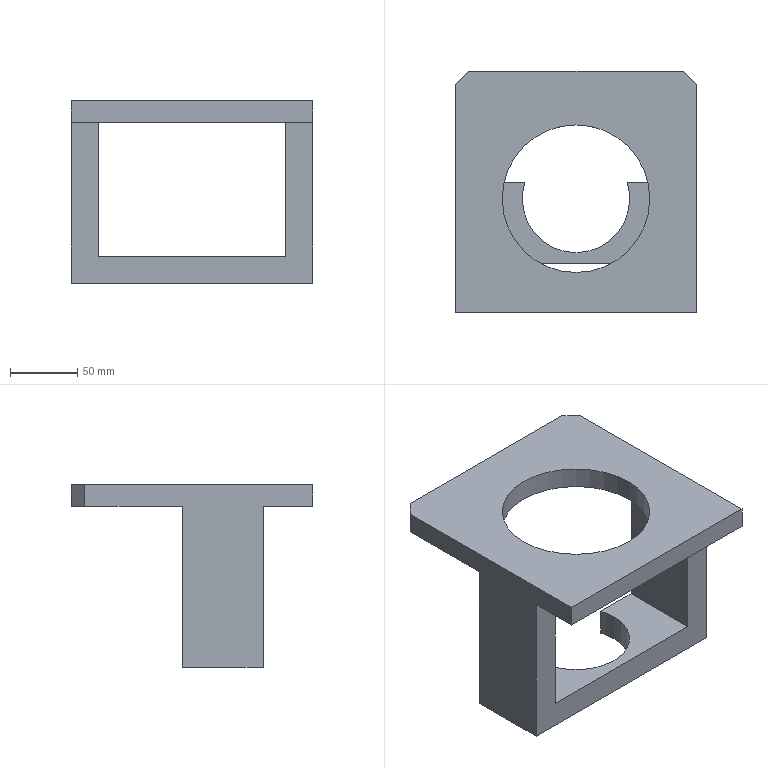Component | SolidWorks | L-Bracket-1 | 1 solid | 20 faces | box 180 x 180 x 136 mm | volume 751573 mm3 | plane 15 | cylinder 5 | commonest cylinder face diameters 80 x3 110 x2
build123d program:
from build123d import *

# Parameters (mm, degrees)
EXTRUDE1_DEPTH      = 90
CHAMFER1_SIZE       = 10
SKETCH3_R           = 55
CUT_EXTRUDE1_DEPTH  = 20
BOSS_EXTRUDE1_DEPTH = 60
SKETCH5_R           = 40
CUT_EXTRUDE2_DEPTH  = 230.87


with BuildPart() as part:
    # Sketch1 → Extrude1 (new, symmetric)
    with BuildSketch(Plane.XY):
        Polygon((0, 0), (0, -18), (16, -18), (16, -4), (16, 162), (0, 162), align=None)
    extrude(amount=EXTRUDE1_DEPTH, both=True)

    # Chamfer1
    chamfer1_edges = [part.edges().sort_by_distance(p)[0] for p in [
        (8, 162, 90),
        (8, 162, -90),
    ]]
    chamfer(chamfer1_edges, length=CHAMFER1_SIZE)

    # Sketch3 → Cut-Extrude1 (cut)
    with BuildSketch(Plane.ZY):
        with Locations((0, 67)):
            Circle(SKETCH3_R)
    extrude(amount=-CUT_EXTRUDE1_DEPTH, mode=Mode.SUBTRACT)

    # Sketch4 → Boss-Extrude1 (add)
    with BuildSketch(Plane.XZ.offset(-19)):
        Polygon((-120, -70), (-120, 70), (-120, 90), (0, 90), (0, 70), (-100, 70), (-100, -70), (0, -70), (0, -90), (-120, -90), align=None)
    extrude(amount=-BOSS_EXTRUDE1_DEPTH)

    # Sketch5 → Cut-Extrude2 (cut, through all)
    with BuildSketch(Plane(origin=(16, 0, 0), x_dir=(0, 0, -1), z_dir=(1, 0, 0))):
        with Locations((0, 67)):
            Circle(SKETCH5_R)
    extrude(amount=-CUT_EXTRUDE2_DEPTH, mode=Mode.SUBTRACT)


solid = part.part

# Placed as in the assembly
solid = solid.moved(Location((5.881, -63.556, 146), (0, -90, 0)))
STEP:
#1=COLOUR_RGB('',0.7922,0.8196,0.9333);
#2=FILL_AREA_STYLE_COLOUR('',#1);
#3=FILL_AREA_STYLE('',(#2));
#4=SURFACE_STYLE_FILL_AREA(#3);
#5=SURFACE_SIDE_STYLE('',(#4));
#6=SURFACE_STYLE_USAGE(.BOTH.,#5);
#7=PRESENTATION_STYLE_ASSIGNMENT((#6));
#8=CARTESIAN_POINT('',(-1.343,0.1356,1.024));
#9=VERTEX_POINT('',#8);
#10=CARTESIAN_POINT('',(1.806,0.1356,1.024));
#11=VERTEX_POINT('',#10);
#12=CARTESIAN_POINT('',(0.2315,0.1356,1.024));
#13=DIRECTION('',(0.,0.,1.));
#14=DIRECTION('',(1.,0.,0.));
#15=AXIS2_PLACEMENT_3D('',#12,#13,#14);
#16=CIRCLE('',#15,1.575);
#17=EDGE_CURVE('',#9,#11,#16,.T.);
#18=ORIENTED_EDGE('',*,*,#17,.F.);
#19=CARTESIAN_POINT('',(-1.343,0.1356,1.811));
#20=VERTEX_POINT('',#19);
#21=CARTESIAN_POINT('',(-1.343,0.1356,1.024));
#22=DIRECTION('',(0.,0.,1.));
#23=VECTOR('',#22,39.37);
#24=LINE('',#21,#23);
#25=EDGE_CURVE('',#9,#20,#24,.T.);
#26=ORIENTED_EDGE('',*,*,#25,.T.);
#27=CARTESIAN_POINT('',(1.806,0.1356,1.811));
#28=VERTEX_POINT('',#27);
#29=CARTESIAN_POINT('',(0.2315,0.1356,1.811));
#30=DIRECTION('',(-0.,0.,1.));
#31=DIRECTION('',(1.,0.,0.));
#32=AXIS2_PLACEMENT_3D('',#29,#30,#31);
#33=CIRCLE('',#32,1.575);
#34=EDGE_CURVE('',#20,#28,#33,.T.);
#35=ORIENTED_EDGE('',*,*,#34,.T.);
#36=CARTESIAN_POINT('',(1.806,0.1356,1.024));
#37=DIRECTION('',(0.,0.,1.));
#38=VECTOR('',#37,39.37);
#39=LINE('',#36,#38);
#40=EDGE_CURVE('',#11,#28,#39,.T.);
#41=ORIENTED_EDGE('',*,*,#40,.F.);
#42=EDGE_LOOP('',(#18,#26,#35,#41));
#43=FACE_OUTER_BOUND('',#42,.T.);
#44=CARTESIAN_POINT('',(0.2315,0.1356,1.024));
#45=DIRECTION('',(0.,0.,1.));
#46=DIRECTION('',(1.,0.,0.));
#47=AXIS2_PLACEMENT_3D('',#44,#45,#46);
#48=CYLINDRICAL_SURFACE('',#47,1.575);
#49=ADVANCED_FACE('',(#43),#48,.F.);
#50=CARTESIAN_POINT('',(1.734,0.608,1.024));
#51=VERTEX_POINT('',#50);
#52=CARTESIAN_POINT('',(0.2315,0.1356,1.024));
#53=DIRECTION('',(0.,0.,1.));
#54=DIRECTION('',(1.,0.,0.));
#55=AXIS2_PLACEMENT_3D('',#52,#53,#54);
#56=CIRCLE('',#55,1.575);
#57=EDGE_CURVE('',#11,#51,#56,.T.);
#58=ORIENTED_EDGE('',*,*,#57,.F.);
#59=ORIENTED_EDGE('',*,*,#40,.T.);
#60=CARTESIAN_POINT('',(1.734,0.608,1.811));
#61=VERTEX_POINT('',#60);
#62=CARTESIAN_POINT('',(0.2315,0.1356,1.811));
#63=DIRECTION('',(-0.,0.,1.));
#64=DIRECTION('',(1.,0.,0.));
#65=AXIS2_PLACEMENT_3D('',#62,#63,#64);
#66=CIRCLE('',#65,1.575);
#67=EDGE_CURVE('',#28,#61,#66,.T.);
#68=ORIENTED_EDGE('',*,*,#67,.T.);
#69=CARTESIAN_POINT('',(1.734,0.608,1.024));
#70=DIRECTION('',(0.,0.,-1.));
#71=VECTOR('',#70,39.37);
#72=LINE('',#69,#71);
#73=EDGE_CURVE('',#61,#51,#72,.T.);
#74=ORIENTED_EDGE('',*,*,#73,.T.);
#75=EDGE_LOOP('',(#58,#59,#68,#74));
#76=FACE_OUTER_BOUND('',#75,.T.);
#77=CARTESIAN_POINT('',(0.2315,0.1356,1.024));
#78=DIRECTION('',(0.,0.,1.));
#79=DIRECTION('',(1.,0.,0.));
#80=AXIS2_PLACEMENT_3D('',#77,#78,#79);
#81=CYLINDRICAL_SURFACE('',#80,1.575);
#82=ADVANCED_FACE('',(#76),#81,.F.);
#83=CARTESIAN_POINT('',(2.397,0.1356,6.378));
#84=VERTEX_POINT('',#83);
#85=CARTESIAN_POINT('',(-1.934,0.1356,6.378));
#86=VERTEX_POINT('',#85);
#87=CARTESIAN_POINT('',(0.2315,0.1356,6.378));
#88=DIRECTION('',(0.,0.,-1.));
#89=DIRECTION('',(-1.,0.,0.));
#90=AXIS2_PLACEMENT_3D('',#87,#88,#89);
#91=CIRCLE('',#90,2.165);
#92=EDGE_CURVE('',#84,#86,#91,.T.);
#93=ORIENTED_EDGE('',*,*,#92,.F.);
#94=CARTESIAN_POINT('',(2.397,0.1356,5.748));
#95=VERTEX_POINT('',#94);
#96=CARTESIAN_POINT('',(2.397,0.1356,6.535));
#97=DIRECTION('',(0.,0.,-1.));
#98=VECTOR('',#97,39.37);
#99=LINE('',#96,#98);
#100=EDGE_CURVE('',#84,#95,#99,.T.);
#101=ORIENTED_EDGE('',*,*,#100,.T.);
#102=CARTESIAN_POINT('',(-1.934,0.1356,5.748));
#103=VERTEX_POINT('',#102);
#104=CARTESIAN_POINT('',(0.2315,0.1356,5.748));
#105=DIRECTION('',(0.,0.,-1.));
#106=DIRECTION('',(-1.,0.,0.));
#107=AXIS2_PLACEMENT_3D('',#104,#105,#106);
#108=CIRCLE('',#107,2.165);
#109=EDGE_CURVE('',#95,#103,#108,.T.);
#110=ORIENTED_EDGE('',*,*,#109,.T.);
#111=CARTESIAN_POINT('',(-1.934,0.1356,6.535));
#112=DIRECTION('',(0.,0.,-1.));
#113=VECTOR('',#112,39.37);
#114=LINE('',#111,#113);
#115=EDGE_CURVE('',#86,#103,#114,.T.);
#116=ORIENTED_EDGE('',*,*,#115,.F.);
#117=EDGE_LOOP('',(#93,#101,#110,#116));
#118=FACE_OUTER_BOUND('',#117,.T.);
#119=CARTESIAN_POINT('',(0.2315,0.1356,6.535));
#120=DIRECTION('',(0.,0.,-1.));
#121=DIRECTION('',(-1.,0.,0.));
#122=AXIS2_PLACEMENT_3D('',#119,#120,#121);
#123=CYLINDRICAL_SURFACE('',#122,2.165);
#124=ADVANCED_FACE('',(#118),#123,.F.);
#125=CARTESIAN_POINT('',(-1.271,0.608,1.024));
#126=VERTEX_POINT('',#125);
#127=CARTESIAN_POINT('',(-1.271,0.608,1.811));
#128=VERTEX_POINT('',#127);
#129=CARTESIAN_POINT('',(-1.271,0.608,1.024));
#130=DIRECTION('',(0.,0.,1.));
#131=VECTOR('',#130,39.37);
#132=LINE('',#129,#131);
#133=EDGE_CURVE('',#126,#128,#132,.T.);
#134=ORIENTED_EDGE('',*,*,#133,.F.);
#135=CARTESIAN_POINT('',(-3.312,0.608,1.024));
#136=VERTEX_POINT('',#135);
#137=CARTESIAN_POINT('',(-3.312,0.608,1.024));
#138=DIRECTION('',(1.,0.,0.));
#139=VECTOR('',#138,39.37);
#140=LINE('',#137,#139);
#141=EDGE_CURVE('',#136,#126,#140,.T.);
#142=ORIENTED_EDGE('',*,*,#141,.F.);
#143=CARTESIAN_POINT('',(-3.312,0.608,5.748));
#144=VERTEX_POINT('',#143);
#145=CARTESIAN_POINT('',(-3.312,0.608,5.748));
#146=DIRECTION('',(0.,0.,-1.));
#147=VECTOR('',#146,39.37);
#148=LINE('',#145,#147);
#149=EDGE_CURVE('',#144,#136,#148,.T.);
#150=ORIENTED_EDGE('',*,*,#149,.F.);
#151=CARTESIAN_POINT('',(-2.524,0.608,5.748));
#152=VERTEX_POINT('',#151);
#153=CARTESIAN_POINT('',(-3.312,0.608,5.748));
#154=DIRECTION('',(-1.,0.,-0.));
#155=VECTOR('',#154,39.37);
#156=LINE('',#153,#155);
#157=EDGE_CURVE('',#152,#144,#156,.T.);
#158=ORIENTED_EDGE('',*,*,#157,.F.);
#159=CARTESIAN_POINT('',(-2.524,0.608,1.811));
#160=VERTEX_POINT('',#159);
#161=CARTESIAN_POINT('',(-2.524,0.608,5.748));
#162=DIRECTION('',(-0.,0.,1.));
#163=VECTOR('',#162,39.37);
#164=LINE('',#161,#163);
#165=EDGE_CURVE('',#160,#152,#164,.T.);
#166=ORIENTED_EDGE('',*,*,#165,.F.);
#167=CARTESIAN_POINT('',(-2.524,0.608,1.811));
#168=DIRECTION('',(-1.,0.,-0.));
#169=VECTOR('',#168,39.37);
#170=LINE('',#167,#169);
#171=EDGE_CURVE('',#128,#160,#170,.T.);
#172=ORIENTED_EDGE('',*,*,#171,.F.);
#173=EDGE_LOOP('',(#134,#142,#150,#158,#166,#172));
#174=FACE_OUTER_BOUND('',#173,.T.);
#175=CARTESIAN_POINT('',(-2.524,0.608,5.748));
#176=DIRECTION('',(0.,1.,0.));
#177=DIRECTION('',(-1.,0.,0.));
#178=AXIS2_PLACEMENT_3D('',#175,#176,#177);
#179=PLANE('',#178);
#180=ADVANCED_FACE('',(#174),#179,.T.);
#181=CARTESIAN_POINT('',(0.2315,0.1356,5.748));
#182=DIRECTION('',(0.,0.,-1.));
#183=DIRECTION('',(-1.,0.,0.));
#184=AXIS2_PLACEMENT_3D('',#181,#182,#183);
#185=CIRCLE('',#184,2.165);
#186=EDGE_CURVE('',#103,#95,#185,.T.);
#187=ORIENTED_EDGE('',*,*,#186,.F.);
#188=ORIENTED_EDGE('',*,*,#109,.F.);
#189=EDGE_LOOP('',(#187,#188));
#190=FACE_BOUND('',#189,.T.);
#191=CARTESIAN_POINT('',(3.775,3.482,5.748));
#192=VERTEX_POINT('',#191);
#193=CARTESIAN_POINT('',(3.775,0.608,5.748));
#194=VERTEX_POINT('',#193);
#195=CARTESIAN_POINT('',(3.775,-2.502,5.748));
#196=DIRECTION('',(0.,-1.,0.));
#197=VECTOR('',#196,39.37);
#198=LINE('',#195,#197);
#199=EDGE_CURVE('',#192,#194,#198,.T.);
#200=ORIENTED_EDGE('',*,*,#199,.T.);
#201=CARTESIAN_POINT('',(2.987,0.608,5.748));
#202=VERTEX_POINT('',#201);
#203=CARTESIAN_POINT('',(3.775,0.608,5.748));
#204=DIRECTION('',(-1.,0.,0.));
#205=VECTOR('',#204,39.37);
#206=LINE('',#203,#205);
#207=EDGE_CURVE('',#194,#202,#206,.T.);
#208=ORIENTED_EDGE('',*,*,#207,.T.);
#209=CARTESIAN_POINT('',(2.987,-1.754,5.748));
#210=VERTEX_POINT('',#209);
#211=CARTESIAN_POINT('',(2.987,0.608,5.748));
#212=DIRECTION('',(0.,-1.,0.));
#213=VECTOR('',#212,39.37);
#214=LINE('',#211,#213);
#215=EDGE_CURVE('',#202,#210,#214,.T.);
#216=ORIENTED_EDGE('',*,*,#215,.T.);
#217=CARTESIAN_POINT('',(3.775,-1.754,5.748));
#218=VERTEX_POINT('',#217);
#219=CARTESIAN_POINT('',(3.775,-1.754,5.748));
#220=DIRECTION('',(-1.,0.,0.));
#221=VECTOR('',#220,39.37);
#222=LINE('',#219,#221);
#223=EDGE_CURVE('',#218,#210,#222,.T.);
#224=ORIENTED_EDGE('',*,*,#223,.F.);
#225=CARTESIAN_POINT('',(3.775,-3.211,5.748));
#226=VERTEX_POINT('',#225);
#227=CARTESIAN_POINT('',(3.775,-2.502,5.748));
#228=DIRECTION('',(0.,-1.,0.));
#229=VECTOR('',#228,39.37);
#230=LINE('',#227,#229);
#231=EDGE_CURVE('',#218,#226,#230,.T.);
#232=ORIENTED_EDGE('',*,*,#231,.T.);
#233=CARTESIAN_POINT('',(-3.312,-3.211,5.748));
#234=VERTEX_POINT('',#233);
#235=CARTESIAN_POINT('',(-3.312,-3.211,5.748));
#236=DIRECTION('',(1.,0.,0.));
#237=VECTOR('',#236,39.37);
#238=LINE('',#235,#237);
#239=EDGE_CURVE('',#234,#226,#238,.T.);
#240=ORIENTED_EDGE('',*,*,#239,.F.);
#241=CARTESIAN_POINT('',(-3.312,-1.754,5.748));
#242=VERTEX_POINT('',#241);
#243=CARTESIAN_POINT('',(-3.312,-2.502,5.748));
#244=DIRECTION('',(0.,-1.,0.));
#245=VECTOR('',#244,39.37);
#246=LINE('',#243,#245);
#247=EDGE_CURVE('',#242,#234,#246,.T.);
#248=ORIENTED_EDGE('',*,*,#247,.F.);
#249=CARTESIAN_POINT('',(-2.524,-1.754,5.748));
#250=VERTEX_POINT('',#249);
#251=CARTESIAN_POINT('',(-3.312,-1.754,5.748));
#252=DIRECTION('',(-1.,0.,-0.));
#253=VECTOR('',#252,39.37);
#254=LINE('',#251,#253);
#255=EDGE_CURVE('',#250,#242,#254,.T.);
#256=ORIENTED_EDGE('',*,*,#255,.F.);
#257=CARTESIAN_POINT('',(-2.524,0.608,5.748));
#258=DIRECTION('',(0.,-1.,0.));
#259=VECTOR('',#258,39.37);
#260=LINE('',#257,#259);
#261=EDGE_CURVE('',#152,#250,#260,.T.);
#262=ORIENTED_EDGE('',*,*,#261,.F.);
#263=ORIENTED_EDGE('',*,*,#157,.T.);
#264=CARTESIAN_POINT('',(-3.312,3.482,5.748));
#265=VERTEX_POINT('',#264);
#266=CARTESIAN_POINT('',(-3.312,-2.502,5.748));
#267=DIRECTION('',(0.,-1.,0.));
#268=VECTOR('',#267,39.37);
#269=LINE('',#266,#268);
#270=EDGE_CURVE('',#265,#144,#269,.T.);
#271=ORIENTED_EDGE('',*,*,#270,.F.);
#272=CARTESIAN_POINT('',(-2.918,3.876,5.748));
#273=VERTEX_POINT('',#272);
#274=CARTESIAN_POINT('',(-3.312,3.482,5.748));
#275=DIRECTION('',(0.7071,0.7071,0.));
#276=VECTOR('',#275,39.37);
#277=LINE('',#274,#276);
#278=EDGE_CURVE('',#265,#273,#277,.T.);
#279=ORIENTED_EDGE('',*,*,#278,.T.);
#280=CARTESIAN_POINT('',(3.381,3.876,5.748));
#281=VERTEX_POINT('',#280);
#282=CARTESIAN_POINT('',(-3.312,3.876,5.748));
#283=DIRECTION('',(1.,0.,0.));
#284=VECTOR('',#283,39.37);
#285=LINE('',#282,#284);
#286=EDGE_CURVE('',#273,#281,#285,.T.);
#287=ORIENTED_EDGE('',*,*,#286,.T.);
#288=CARTESIAN_POINT('',(3.381,3.876,5.748));
#289=DIRECTION('',(0.7071,-0.7071,0.));
#290=VECTOR('',#289,39.37);
#291=LINE('',#288,#290);
#292=EDGE_CURVE('',#281,#192,#291,.T.);
#293=ORIENTED_EDGE('',*,*,#292,.T.);
#294=EDGE_LOOP('',(#200,#208,#216,#224,#232,#240,#248,#256,#262,#263,#271,#279,#287,#293));
#295=FACE_OUTER_BOUND('',#294,.T.);
#296=CARTESIAN_POINT('',(-3.312,-2.502,5.748));
#297=DIRECTION('',(0.,0.,1.));
#298=DIRECTION('',(1.,0.,0.));
#299=AXIS2_PLACEMENT_3D('',#296,#297,#298);
#300=PLANE('',#299);
#301=ADVANCED_FACE('',(#190,#295),#300,.F.);
#302=CARTESIAN_POINT('',(3.775,-3.211,6.378));
#303=VERTEX_POINT('',#302);
#304=CARTESIAN_POINT('',(3.775,-3.211,5.748));
#305=DIRECTION('',(0.,0.,1.));
#306=VECTOR('',#305,39.37);
#307=LINE('',#304,#306);
#308=EDGE_CURVE('',#226,#303,#307,.T.);
#309=ORIENTED_EDGE('',*,*,#308,.T.);
#310=CARTESIAN_POINT('',(-3.312,-3.211,6.378));
#311=VERTEX_POINT('',#310);
#312=CARTESIAN_POINT('',(-3.312,-3.211,6.378));
#313=DIRECTION('',(1.,0.,0.));
#314=VECTOR('',#313,39.37);
#315=LINE('',#312,#314);
#316=EDGE_CURVE('',#311,#303,#315,.T.);
#317=ORIENTED_EDGE('',*,*,#316,.F.);
#318=CARTESIAN_POINT('',(-3.312,-3.211,5.748));
#319=DIRECTION('',(0.,0.,1.));
#320=VECTOR('',#319,39.37);
#321=LINE('',#318,#320);
#322=EDGE_CURVE('',#234,#311,#321,.T.);
#323=ORIENTED_EDGE('',*,*,#322,.F.);
#324=ORIENTED_EDGE('',*,*,#239,.T.);
#325=EDGE_LOOP('',(#309,#317,#323,#324));
#326=FACE_OUTER_BOUND('',#325,.T.);
#327=CARTESIAN_POINT('',(-3.312,-3.211,5.748));
#328=DIRECTION('',(0.,1.,0.));
#329=DIRECTION('',(-1.,0.,0.));
#330=AXIS2_PLACEMENT_3D('',#327,#328,#329);
#331=PLANE('',#330);
#332=ADVANCED_FACE('',(#326),#331,.F.);
#333=CARTESIAN_POINT('',(0.2315,0.1356,6.378));
#334=DIRECTION('',(0.,0.,-1.));
#335=DIRECTION('',(-1.,0.,0.));
#336=AXIS2_PLACEMENT_3D('',#333,#334,#335);
#337=CIRCLE('',#336,2.165);
#338=EDGE_CURVE('',#86,#84,#337,.T.);
#339=ORIENTED_EDGE('',*,*,#338,.T.);
#340=ORIENTED_EDGE('',*,*,#92,.T.);
#341=EDGE_LOOP('',(#339,#340));
#342=FACE_BOUND('',#341,.T.);
#343=CARTESIAN_POINT('',(3.775,3.482,6.378));
#344=VERTEX_POINT('',#343);
#345=CARTESIAN_POINT('',(3.775,-2.66,6.378));
#346=DIRECTION('',(0.,1.,0.));
#347=VECTOR('',#346,39.37);
#348=LINE('',#345,#347);
#349=EDGE_CURVE('',#303,#344,#348,.T.);
#350=ORIENTED_EDGE('',*,*,#349,.T.);
#351=CARTESIAN_POINT('',(3.381,3.876,6.378));
#352=VERTEX_POINT('',#351);
#353=CARTESIAN_POINT('',(3.381,3.876,6.378));
#354=DIRECTION('',(-0.7071,0.7071,0.));
#355=VECTOR('',#354,39.37);
#356=LINE('',#353,#355);
#357=EDGE_CURVE('',#344,#352,#356,.T.);
#358=ORIENTED_EDGE('',*,*,#357,.T.);
#359=CARTESIAN_POINT('',(-2.918,3.876,6.378));
#360=VERTEX_POINT('',#359);
#361=CARTESIAN_POINT('',(-3.312,3.876,6.378));
#362=DIRECTION('',(1.,0.,0.));
#363=VECTOR('',#362,39.37);
#364=LINE('',#361,#363);
#365=EDGE_CURVE('',#360,#352,#364,.T.);
#366=ORIENTED_EDGE('',*,*,#365,.F.);
#367=CARTESIAN_POINT('',(-3.312,3.482,6.378));
#368=VERTEX_POINT('',#367);
#369=CARTESIAN_POINT('',(-3.312,3.482,6.378));
#370=DIRECTION('',(-0.7071,-0.7071,0.));
#371=VECTOR('',#370,39.37);
#372=LINE('',#369,#371);
#373=EDGE_CURVE('',#360,#368,#372,.T.);
#374=ORIENTED_EDGE('',*,*,#373,.T.);
#375=CARTESIAN_POINT('',(-3.312,-2.66,6.378));
#376=DIRECTION('',(0.,1.,0.));
#377=VECTOR('',#376,39.37);
#378=LINE('',#375,#377);
#379=EDGE_CURVE('',#311,#368,#378,.T.);
#380=ORIENTED_EDGE('',*,*,#379,.F.);
#381=ORIENTED_EDGE('',*,*,#316,.T.);
#382=EDGE_LOOP('',(#350,#358,#366,#374,#380,#381));
#383=FACE_OUTER_BOUND('',#382,.T.);
#384=CARTESIAN_POINT('',(-3.312,-2.66,6.378));
#385=DIRECTION('',(0.,0.,-1.));
#386=DIRECTION('',(-1.,0.,0.));
#387=AXIS2_PLACEMENT_3D('',#384,#385,#386);
#388=PLANE('',#387);
#389=ADVANCED_FACE('',(#342,#383),#388,.F.);
#390=ORIENTED_EDGE('',*,*,#365,.T.);
#391=CARTESIAN_POINT('',(3.381,3.876,5.748));
#392=DIRECTION('',(0.,0.,-1.));
#393=VECTOR('',#392,39.37);
#394=LINE('',#391,#393);
#395=EDGE_CURVE('',#352,#281,#394,.T.);
#396=ORIENTED_EDGE('',*,*,#395,.T.);
#397=ORIENTED_EDGE('',*,*,#286,.F.);
#398=CARTESIAN_POINT('',(-2.918,3.876,5.748));
#399=DIRECTION('',(0.,0.,1.));
#400=VECTOR('',#399,39.37);
#401=LINE('',#398,#400);
#402=EDGE_CURVE('',#273,#360,#401,.T.);
#403=ORIENTED_EDGE('',*,*,#402,.T.);
#404=EDGE_LOOP('',(#390,#396,#397,#403));
#405=FACE_OUTER_BOUND('',#404,.T.);
#406=CARTESIAN_POINT('',(-3.312,3.876,5.748));
#407=DIRECTION('',(0.,-1.,0.));
#408=DIRECTION('',(1.,0.,0.));
#409=AXIS2_PLACEMENT_3D('',#406,#407,#408);
#410=PLANE('',#409);
#411=ADVANCED_FACE('',(#405),#410,.F.);
#412=ORIENTED_EDGE('',*,*,#379,.T.);
#413=CARTESIAN_POINT('',(-3.312,3.482,5.748));
#414=DIRECTION('',(0.,0.,-1.));
#415=VECTOR('',#414,39.37);
#416=LINE('',#413,#415);
#417=EDGE_CURVE('',#368,#265,#416,.T.);
#418=ORIENTED_EDGE('',*,*,#417,.T.);
#419=ORIENTED_EDGE('',*,*,#270,.T.);
#420=ORIENTED_EDGE('',*,*,#149,.T.);
#421=CARTESIAN_POINT('',(-3.312,-1.754,1.024));
#422=VERTEX_POINT('',#421);
#423=CARTESIAN_POINT('',(-3.312,0.608,1.024));
#424=DIRECTION('',(0.,-1.,0.));
#425=VECTOR('',#424,39.37);
#426=LINE('',#423,#425);
#427=EDGE_CURVE('',#136,#422,#426,.T.);
#428=ORIENTED_EDGE('',*,*,#427,.T.);
#429=CARTESIAN_POINT('',(-3.312,-1.754,5.748));
#430=DIRECTION('',(0.,0.,-1.));
#431=VECTOR('',#430,39.37);
#432=LINE('',#429,#431);
#433=EDGE_CURVE('',#242,#422,#432,.T.);
#434=ORIENTED_EDGE('',*,*,#433,.F.);
#435=ORIENTED_EDGE('',*,*,#247,.T.);
#436=ORIENTED_EDGE('',*,*,#322,.T.);
#437=EDGE_LOOP('',(#412,#418,#419,#420,#428,#434,#435,#436));
#438=FACE_OUTER_BOUND('',#437,.T.);
#439=CARTESIAN_POINT('',(-3.312,3.876,5.748));
#440=DIRECTION('',(1.,0.,0.));
#441=DIRECTION('',(0.,0.,-1.));
#442=AXIS2_PLACEMENT_3D('',#439,#440,#441);
#443=PLANE('',#442);
#444=ADVANCED_FACE('',(#438),#443,.F.);
#445=ORIENTED_EDGE('',*,*,#199,.F.);
#446=CARTESIAN_POINT('',(3.775,3.482,6.378));
#447=DIRECTION('',(0.,0.,1.));
#448=VECTOR('',#447,39.37);
#449=LINE('',#446,#448);
#450=EDGE_CURVE('',#192,#344,#449,.T.);
#451=ORIENTED_EDGE('',*,*,#450,.T.);
#452=ORIENTED_EDGE('',*,*,#349,.F.);
#453=ORIENTED_EDGE('',*,*,#308,.F.);
#454=ORIENTED_EDGE('',*,*,#231,.F.);
#455=CARTESIAN_POINT('',(3.775,-1.754,1.024));
#456=VERTEX_POINT('',#455);
#457=CARTESIAN_POINT('',(3.775,-1.754,5.748));
#458=DIRECTION('',(-0.,0.,1.));
#459=VECTOR('',#458,39.37);
#460=LINE('',#457,#459);
#461=EDGE_CURVE('',#456,#218,#460,.T.);
#462=ORIENTED_EDGE('',*,*,#461,.F.);
#463=CARTESIAN_POINT('',(3.775,0.608,1.024));
#464=VERTEX_POINT('',#463);
#465=CARTESIAN_POINT('',(3.775,0.608,1.024));
#466=DIRECTION('',(0.,-1.,0.));
#467=VECTOR('',#466,39.37);
#468=LINE('',#465,#467);
#469=EDGE_CURVE('',#464,#456,#468,.T.);
#470=ORIENTED_EDGE('',*,*,#469,.F.);
#471=CARTESIAN_POINT('',(3.775,0.608,5.748));
#472=DIRECTION('',(-0.,0.,1.));
#473=VECTOR('',#472,39.37);
#474=LINE('',#471,#473);
#475=EDGE_CURVE('',#464,#194,#474,.T.);
#476=ORIENTED_EDGE('',*,*,#475,.T.);
#477=EDGE_LOOP('',(#445,#451,#452,#453,#454,#462,#470,#476));
#478=FACE_OUTER_BOUND('',#477,.T.);
#479=CARTESIAN_POINT('',(3.775,3.876,5.748));
#480=DIRECTION('',(1.,0.,0.));
#481=DIRECTION('',(0.,0.,-1.));
#482=AXIS2_PLACEMENT_3D('',#479,#480,#481);
#483=PLANE('',#482);
#484=ADVANCED_FACE('',(#478),#483,.T.);
#485=ORIENTED_EDGE('',*,*,#357,.F.);
#486=ORIENTED_EDGE('',*,*,#450,.F.);
#487=ORIENTED_EDGE('',*,*,#292,.F.);
#488=ORIENTED_EDGE('',*,*,#395,.F.);
#489=EDGE_LOOP('',(#485,#486,#487,#488));
#490=FACE_OUTER_BOUND('',#489,.T.);
#491=CARTESIAN_POINT('',(3.381,3.876,5.748));
#492=DIRECTION('',(0.7071,0.7071,0.));
#493=DIRECTION('',(-0.7071,0.7071,0.));
#494=AXIS2_PLACEMENT_3D('',#491,#492,#493);
#495=PLANE('',#494);
#496=ADVANCED_FACE('',(#490),#495,.T.);
#497=ORIENTED_EDGE('',*,*,#373,.F.);
#498=ORIENTED_EDGE('',*,*,#402,.F.);
#499=ORIENTED_EDGE('',*,*,#278,.F.);
#500=ORIENTED_EDGE('',*,*,#417,.F.);
#501=EDGE_LOOP('',(#497,#498,#499,#500));
#502=FACE_OUTER_BOUND('',#501,.T.);
#503=CARTESIAN_POINT('',(-3.312,3.482,5.748));
#504=DIRECTION('',(0.7071,-0.7071,0.));
#505=DIRECTION('',(0.7071,0.7071,0.));
#506=AXIS2_PLACEMENT_3D('',#503,#504,#505);
#507=PLANE('',#506);
#508=ADVANCED_FACE('',(#502),#507,.F.);
#509=ORIENTED_EDGE('',*,*,#100,.F.);
#510=ORIENTED_EDGE('',*,*,#338,.F.);
#511=ORIENTED_EDGE('',*,*,#115,.T.);
#512=ORIENTED_EDGE('',*,*,#186,.T.);
#513=EDGE_LOOP('',(#509,#510,#511,#512));
#514=FACE_OUTER_BOUND('',#513,.T.);
#515=CARTESIAN_POINT('',(0.2315,0.1356,6.535));
#516=DIRECTION('',(0.,0.,-1.));
#517=DIRECTION('',(-1.,0.,0.));
#518=AXIS2_PLACEMENT_3D('',#515,#516,#517);
#519=CYLINDRICAL_SURFACE('',#518,2.165);
#520=ADVANCED_FACE('',(#514),#519,.F.);
#521=CARTESIAN_POINT('',(-2.524,-1.754,1.811));
#522=VERTEX_POINT('',#521);
#523=CARTESIAN_POINT('',(-2.524,-1.754,5.748));
#524=DIRECTION('',(-0.,0.,1.));
#525=VECTOR('',#524,39.37);
#526=LINE('',#523,#525);
#527=EDGE_CURVE('',#522,#250,#526,.T.);
#528=ORIENTED_EDGE('',*,*,#527,.F.);
#529=CARTESIAN_POINT('',(-2.524,0.608,1.811));
#530=DIRECTION('',(0.,-1.,0.));
#531=VECTOR('',#530,39.37);
#532=LINE('',#529,#531);
#533=EDGE_CURVE('',#160,#522,#532,.T.);
#534=ORIENTED_EDGE('',*,*,#533,.F.);
#535=ORIENTED_EDGE('',*,*,#165,.T.);
#536=ORIENTED_EDGE('',*,*,#261,.T.);
#537=EDGE_LOOP('',(#528,#534,#535,#536));
#538=FACE_OUTER_BOUND('',#537,.T.);
#539=CARTESIAN_POINT('',(-2.524,0.608,5.748));
#540=DIRECTION('',(1.,0.,0.));
#541=DIRECTION('',(0.,0.,-1.));
#542=AXIS2_PLACEMENT_3D('',#539,#540,#541);
#543=PLANE('',#542);
#544=ADVANCED_FACE('',(#538),#543,.T.);
#545=CARTESIAN_POINT('',(0.2315,0.1356,1.811));
#546=DIRECTION('',(-0.,0.,1.));
#547=DIRECTION('',(1.,0.,0.));
#548=AXIS2_PLACEMENT_3D('',#545,#546,#547);
#549=CIRCLE('',#548,1.575);
#550=EDGE_CURVE('',#128,#20,#549,.T.);
#551=ORIENTED_EDGE('',*,*,#550,.F.);
#552=ORIENTED_EDGE('',*,*,#171,.T.);
#553=ORIENTED_EDGE('',*,*,#533,.T.);
#554=CARTESIAN_POINT('',(2.987,-1.754,1.811));
#555=VERTEX_POINT('',#554);
#556=CARTESIAN_POINT('',(-2.524,-1.754,1.811));
#557=DIRECTION('',(-1.,0.,-0.));
#558=VECTOR('',#557,39.37);
#559=LINE('',#556,#558);
#560=EDGE_CURVE('',#555,#522,#559,.T.);
#561=ORIENTED_EDGE('',*,*,#560,.F.);
#562=CARTESIAN_POINT('',(2.987,0.608,1.811));
#563=VERTEX_POINT('',#562);
#564=CARTESIAN_POINT('',(2.987,0.608,1.811));
#565=DIRECTION('',(0.,-1.,0.));
#566=VECTOR('',#565,39.37);
#567=LINE('',#564,#566);
#568=EDGE_CURVE('',#563,#555,#567,.T.);
#569=ORIENTED_EDGE('',*,*,#568,.F.);
#570=CARTESIAN_POINT('',(-2.524,0.608,1.811));
#571=DIRECTION('',(-1.,0.,-0.));
#572=VECTOR('',#571,39.37);
#573=LINE('',#570,#572);
#574=EDGE_CURVE('',#563,#61,#573,.T.);
#575=ORIENTED_EDGE('',*,*,#574,.T.);
#576=ORIENTED_EDGE('',*,*,#67,.F.);
#577=ORIENTED_EDGE('',*,*,#34,.F.);
#578=EDGE_LOOP('',(#551,#552,#553,#561,#569,#575,#576,#577));
#579=FACE_OUTER_BOUND('',#578,.T.);
#580=CARTESIAN_POINT('',(-2.524,0.608,1.811));
#581=DIRECTION('',(-0.,0.,1.));
#582=DIRECTION('',(1.,0.,0.));
#583=AXIS2_PLACEMENT_3D('',#580,#581,#582);
#584=PLANE('',#583);
#585=ADVANCED_FACE('',(#579),#584,.T.);
#586=CARTESIAN_POINT('',(2.987,-1.754,5.748));
#587=DIRECTION('',(0.,0.,-1.));
#588=VECTOR('',#587,39.37);
#589=LINE('',#586,#588);
#590=EDGE_CURVE('',#210,#555,#589,.T.);
#591=ORIENTED_EDGE('',*,*,#590,.F.);
#592=ORIENTED_EDGE('',*,*,#215,.F.);
#593=CARTESIAN_POINT('',(2.987,0.608,5.748));
#594=DIRECTION('',(0.,0.,-1.));
#595=VECTOR('',#594,39.37);
#596=LINE('',#593,#595);
#597=EDGE_CURVE('',#202,#563,#596,.T.);
#598=ORIENTED_EDGE('',*,*,#597,.T.);
#599=ORIENTED_EDGE('',*,*,#568,.T.);
#600=EDGE_LOOP('',(#591,#592,#598,#599));
#601=FACE_OUTER_BOUND('',#600,.T.);
#602=CARTESIAN_POINT('',(2.987,0.608,5.748));
#603=DIRECTION('',(-1.,0.,-0.));
#604=DIRECTION('',(-0.,0.,1.));
#605=AXIS2_PLACEMENT_3D('',#602,#603,#604);
#606=PLANE('',#605);
#607=ADVANCED_FACE('',(#601),#606,.T.);
#608=CARTESIAN_POINT('',(0.2315,0.1356,1.024));
#609=DIRECTION('',(0.,0.,1.));
#610=DIRECTION('',(1.,0.,0.));
#611=AXIS2_PLACEMENT_3D('',#608,#609,#610);
#612=CIRCLE('',#611,1.575);
#613=EDGE_CURVE('',#126,#9,#612,.T.);
#614=ORIENTED_EDGE('',*,*,#613,.T.);
#615=ORIENTED_EDGE('',*,*,#17,.T.);
#616=ORIENTED_EDGE('',*,*,#57,.T.);
#617=CARTESIAN_POINT('',(-3.312,0.608,1.024));
#618=DIRECTION('',(1.,0.,0.));
#619=VECTOR('',#618,39.37);
#620=LINE('',#617,#619);
#621=EDGE_CURVE('',#51,#464,#620,.T.);
#622=ORIENTED_EDGE('',*,*,#621,.T.);
#623=ORIENTED_EDGE('',*,*,#469,.T.);
#624=CARTESIAN_POINT('',(3.775,-1.754,1.024));
#625=DIRECTION('',(1.,0.,0.));
#626=VECTOR('',#625,39.37);
#627=LINE('',#624,#626);
#628=EDGE_CURVE('',#422,#456,#627,.T.);
#629=ORIENTED_EDGE('',*,*,#628,.F.);
#630=ORIENTED_EDGE('',*,*,#427,.F.);
#631=ORIENTED_EDGE('',*,*,#141,.T.);
#632=EDGE_LOOP('',(#614,#615,#616,#622,#623,#629,#630,#631));
#633=FACE_OUTER_BOUND('',#632,.T.);
#634=CARTESIAN_POINT('',(3.775,0.608,1.024));
#635=DIRECTION('',(0.,0.,-1.));
#636=DIRECTION('',(-1.,0.,0.));
#637=AXIS2_PLACEMENT_3D('',#634,#635,#636);
#638=PLANE('',#637);
#639=ADVANCED_FACE('',(#633),#638,.T.);
#640=ORIENTED_EDGE('',*,*,#73,.F.);
#641=ORIENTED_EDGE('',*,*,#574,.F.);
#642=ORIENTED_EDGE('',*,*,#597,.F.);
#643=ORIENTED_EDGE('',*,*,#207,.F.);
#644=ORIENTED_EDGE('',*,*,#475,.F.);
#645=ORIENTED_EDGE('',*,*,#621,.F.);
#646=EDGE_LOOP('',(#640,#641,#642,#643,#644,#645));
#647=FACE_OUTER_BOUND('',#646,.T.);
#648=CARTESIAN_POINT('',(-2.524,0.608,5.748));
#649=DIRECTION('',(0.,1.,0.));
#650=DIRECTION('',(-1.,0.,0.));
#651=AXIS2_PLACEMENT_3D('',#648,#649,#650);
#652=PLANE('',#651);
#653=ADVANCED_FACE('',(#647),#652,.T.);
#654=ORIENTED_EDGE('',*,*,#255,.T.);
#655=ORIENTED_EDGE('',*,*,#433,.T.);
#656=ORIENTED_EDGE('',*,*,#628,.T.);
#657=ORIENTED_EDGE('',*,*,#461,.T.);
#658=ORIENTED_EDGE('',*,*,#223,.T.);
#659=ORIENTED_EDGE('',*,*,#590,.T.);
#660=ORIENTED_EDGE('',*,*,#560,.T.);
#661=ORIENTED_EDGE('',*,*,#527,.T.);
#662=EDGE_LOOP('',(#654,#655,#656,#657,#658,#659,#660,#661));
#663=FACE_OUTER_BOUND('',#662,.T.);
#664=CARTESIAN_POINT('',(-2.524,-1.754,5.748));
#665=DIRECTION('',(0.,1.,0.));
#666=DIRECTION('',(-1.,0.,0.));
#667=AXIS2_PLACEMENT_3D('',#664,#665,#666);
#668=PLANE('',#667);
#669=ADVANCED_FACE('',(#663),#668,.F.);
#670=ORIENTED_EDGE('',*,*,#25,.F.);
#671=ORIENTED_EDGE('',*,*,#613,.F.);
#672=ORIENTED_EDGE('',*,*,#133,.T.);
#673=ORIENTED_EDGE('',*,*,#550,.T.);
#674=EDGE_LOOP('',(#670,#671,#672,#673));
#675=FACE_OUTER_BOUND('',#674,.T.);
#676=CARTESIAN_POINT('',(0.2315,0.1356,1.024));
#677=DIRECTION('',(0.,0.,1.));
#678=DIRECTION('',(1.,0.,0.));
#679=AXIS2_PLACEMENT_3D('',#676,#677,#678);
#680=CYLINDRICAL_SURFACE('',#679,1.575);
#681=ADVANCED_FACE('',(#675),#680,.F.);
#682=CLOSED_SHELL('',(#49,#82,#124,#180,#301,#332,#389,#411,#444,#484,#496,#508,#520,#544,#585,#607,#639,#653,#669,#681));
#683=MANIFOLD_SOLID_BREP('',#682);
#684=STYLED_ITEM('',(#7),#683);
#685=(LENGTH_UNIT()NAMED_UNIT(*)SI_UNIT($,.METRE.));
#686=LENGTH_MEASURE_WITH_UNIT(LENGTH_MEASURE(0.0254),#685);
#687=DIMENSIONAL_EXPONENTS(1.,0.,0.,0.,0.,0.,0.);
#688=(CONVERSION_BASED_UNIT('',#686)LENGTH_UNIT()NAMED_UNIT(#687));
#689=UNCERTAINTY_MEASURE_WITH_UNIT(LENGTH_MEASURE(0.00001),#688,'','');
#690=(NAMED_UNIT(*)PLANE_ANGLE_UNIT()SI_UNIT($,.RADIAN.));
#691=(NAMED_UNIT(*)SI_UNIT($,.STERADIAN.)SOLID_ANGLE_UNIT());
#692=(GEOMETRIC_REPRESENTATION_CONTEXT(3)GLOBAL_UNCERTAINTY_ASSIGNED_CONTEXT((#689))GLOBAL_UNIT_ASSIGNED_CONTEXT((#688,#690,#691))REPRESENTATION_CONTEXT('',''));
#693=MECHANICAL_DESIGN_GEOMETRIC_PRESENTATION_REPRESENTATION('',(#684),#692);
#694=PRESENTATION_LAYER_ASSIGNMENT('','',(#684));
#695=CARTESIAN_POINT('',(0.,0.,0.));
#696=DIRECTION('',(0.,0.,1.));
#697=DIRECTION('',(1.,0.,0.));
#698=AXIS2_PLACEMENT_3D('',#695,#696,#697);
#699=(LENGTH_UNIT()NAMED_UNIT(*)SI_UNIT($,.METRE.));
#700=LENGTH_MEASURE_WITH_UNIT(LENGTH_MEASURE(0.0254),#699);
#701=DIMENSIONAL_EXPONENTS(1.,0.,0.,0.,0.,0.,0.);
#702=(CONVERSION_BASED_UNIT('',#700)LENGTH_UNIT()NAMED_UNIT(#701));
#703=UNCERTAINTY_MEASURE_WITH_UNIT(LENGTH_MEASURE(0.00001),#702,'','');
#704=(NAMED_UNIT(*)PLANE_ANGLE_UNIT()SI_UNIT($,.RADIAN.));
#705=(NAMED_UNIT(*)SI_UNIT($,.STERADIAN.)SOLID_ANGLE_UNIT());
#706=(GEOMETRIC_REPRESENTATION_CONTEXT(3)GLOBAL_UNCERTAINTY_ASSIGNED_CONTEXT((#703))GLOBAL_UNIT_ASSIGNED_CONTEXT((#702,#704,#705))REPRESENTATION_CONTEXT('',''));
#707=ADVANCED_BREP_SHAPE_REPRESENTATION('',(#683,#698),#706);